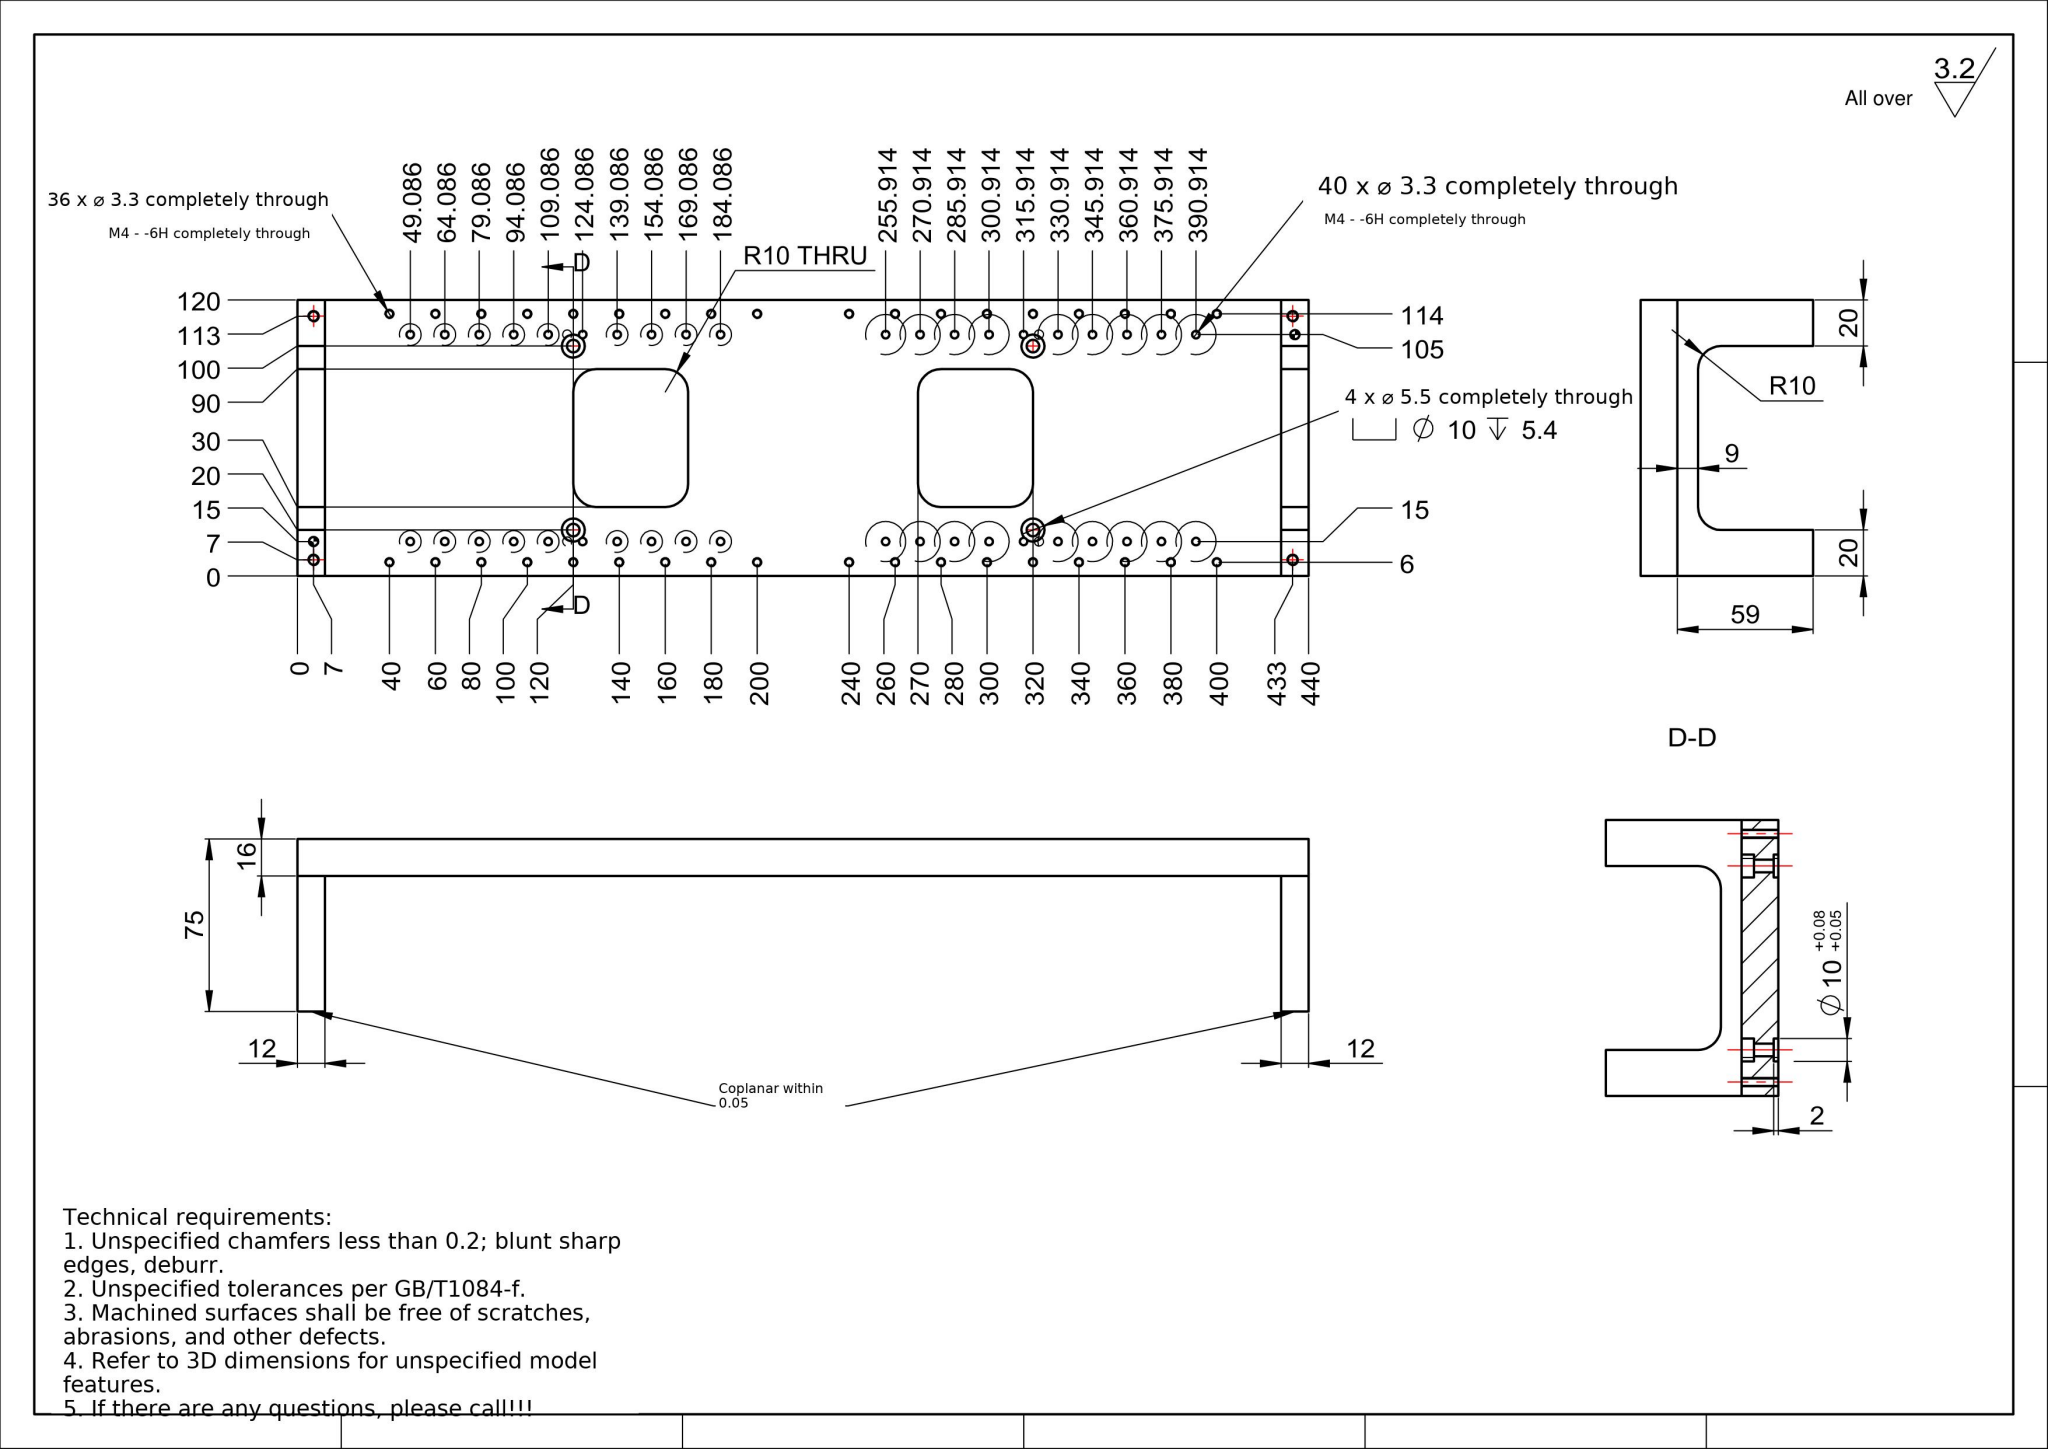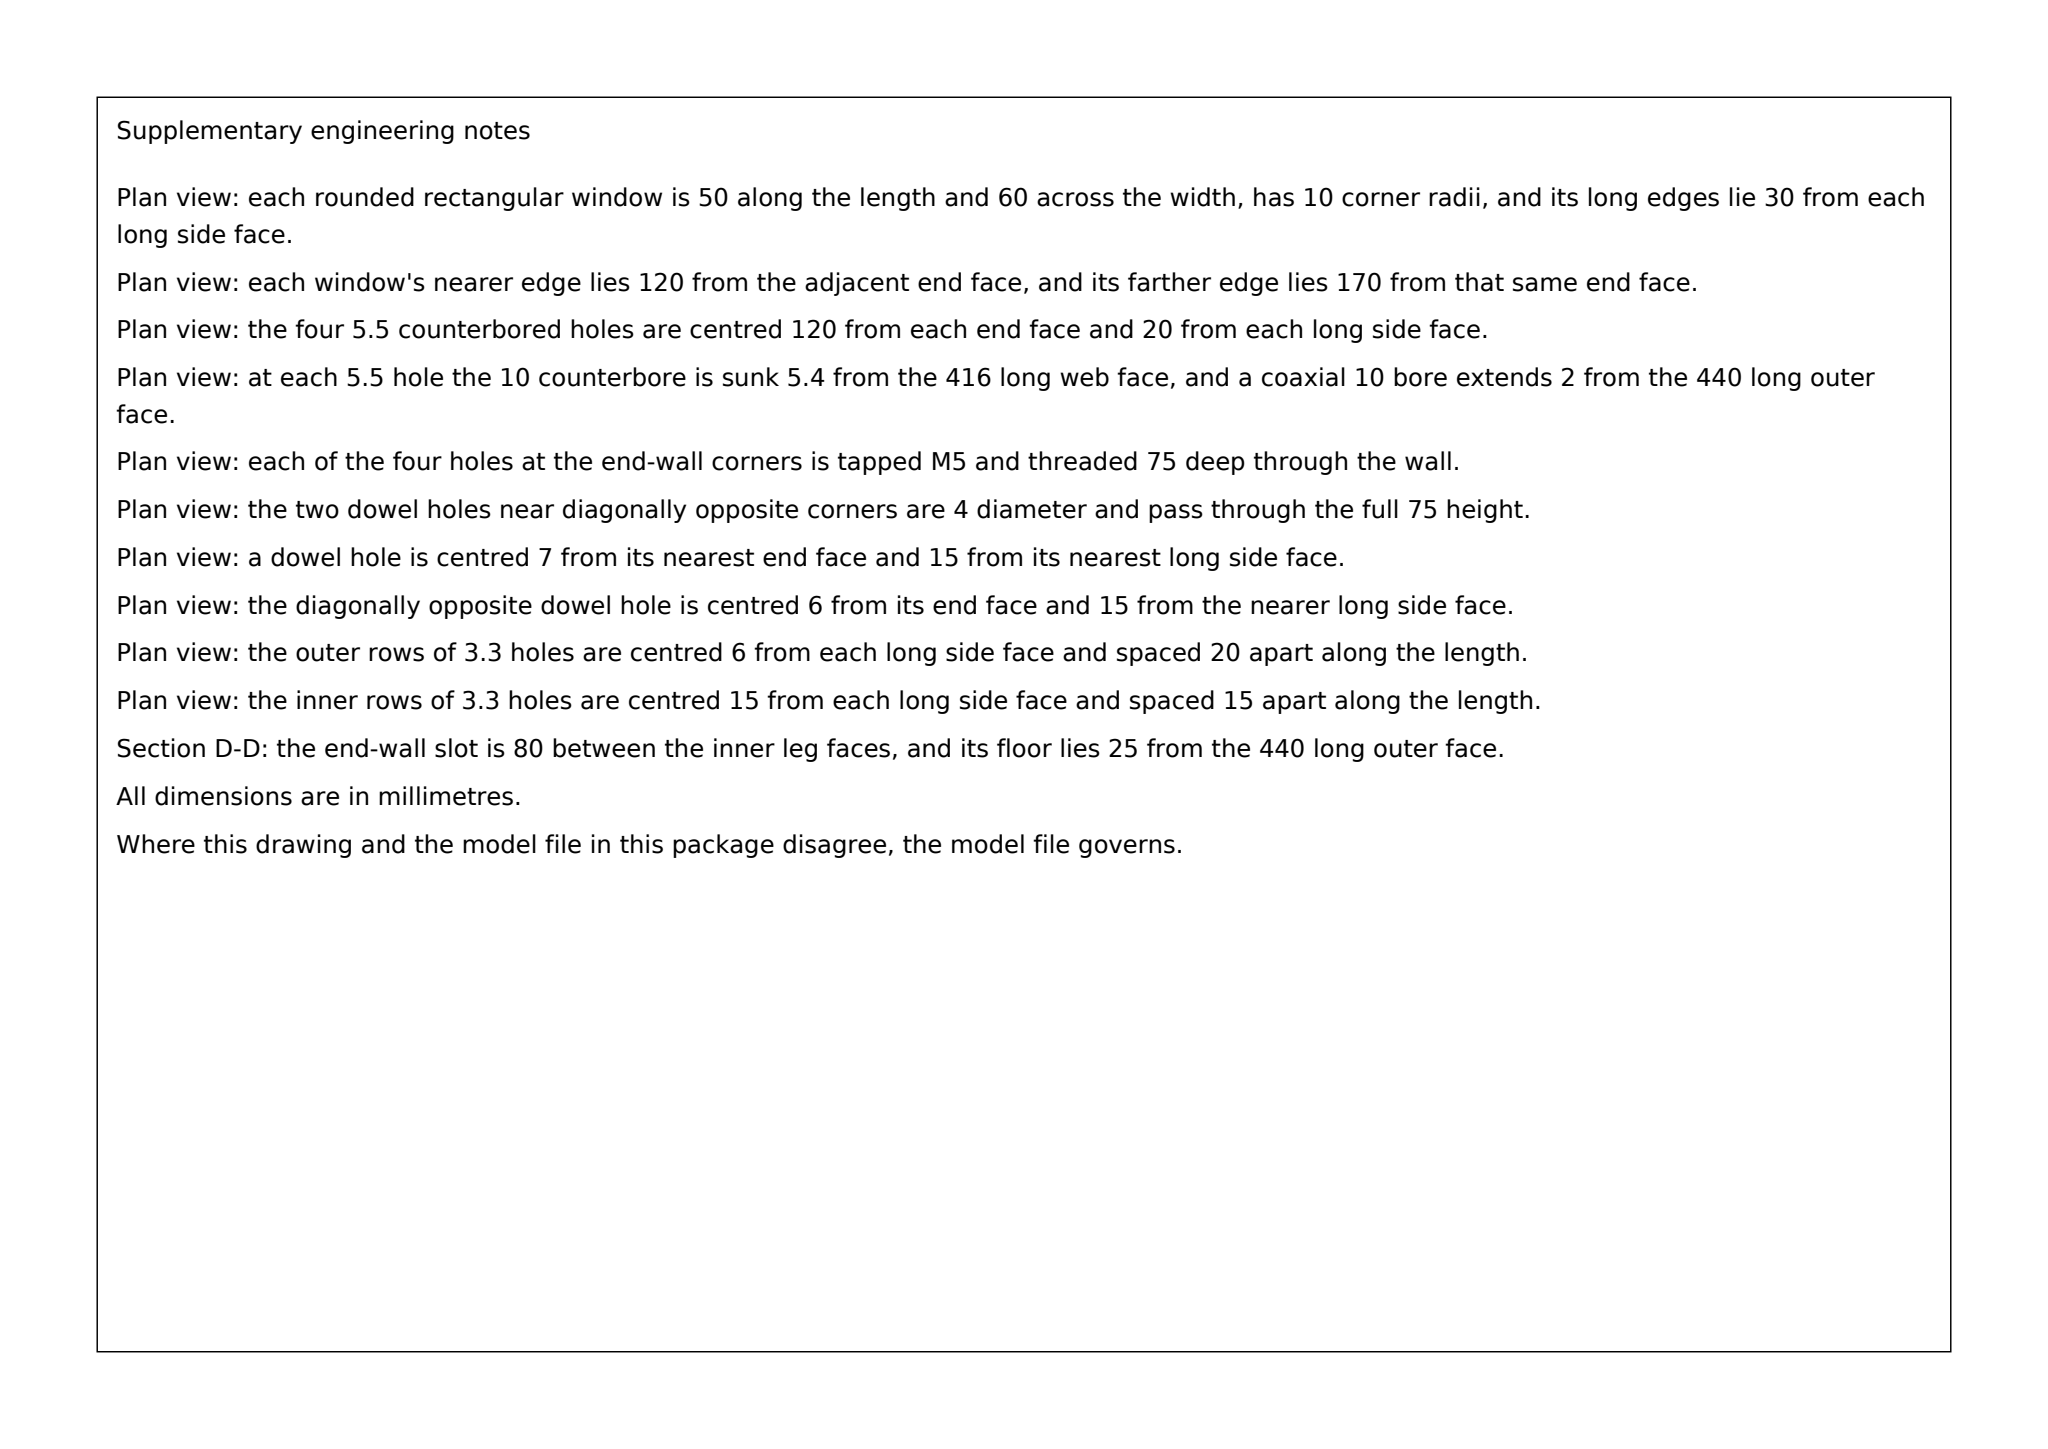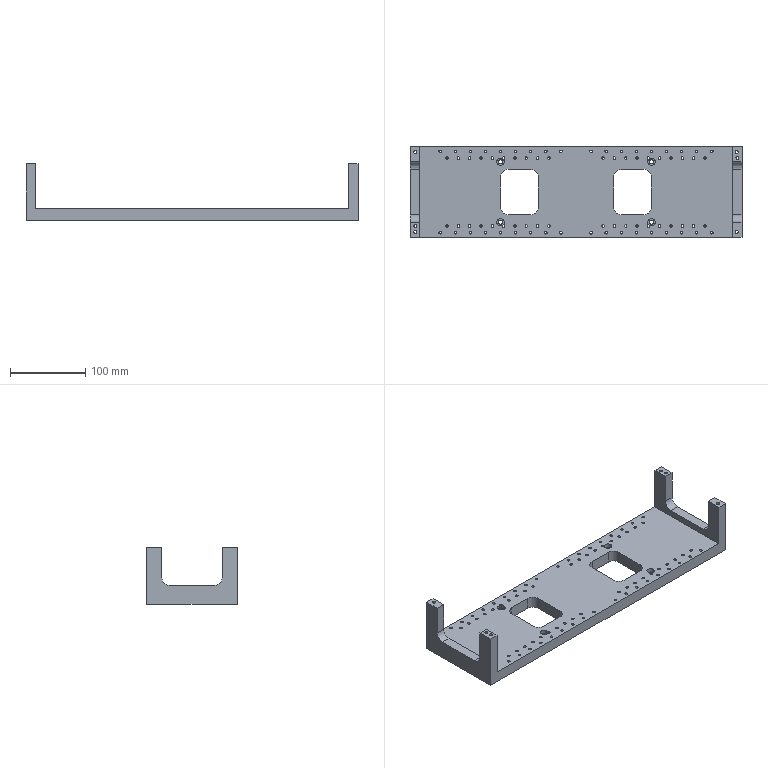Part | SolidWorks | mm | 1 solid | 242 faces | box 440 x 120 x 75 mm | volume 806918 mm3 | cylinder 208 | plane 34 | commonest cylinder face diameters 3.3 x152 10 x24 20 x12 5.5 x8 4.2 x8 4 x4
Drawing notes:
4X Ø4.2 THRU (full depth 75): two holes at x = 7, y = 7 and x = 7, y = 113, measured from the lower-left corner of the part (x0, y0). | from the solid: cylinders[4.2,z,[7.0,7.0],75.0] and cylinders[4.2,z,[7.0,113.0],75.0]
2X Ø4 THRU (full depth 75): one at x = 7, y = 15 and one at x = 434, y = 105 from the lower-left corner (x0, y0). | from the solid: cylinders[4.0,z,[7.0,15.0],75.0] and cylinders[4.0,z,[434.0,105.0],75.0]
R10 THRU pocket (left): pocket walls at x = 120 and x = 170 from the left end face (x = 0); right pocket walls at x = 270 and x = 320. | from the solid: axis_planes[x,120.0], [x,170.0], [x,270.0], [x,320.0]
4X Ø10 +0.08/+0.05 bore DP 2 deep, machined from the z = 0 face (opposite the Ø10 DP 5.4 counterbore face), coaxial with the 4X Ø5.5 THRU holes; counterbore floor at z = 10.6 from the z = 0 face. | from the solid: axis_planes[z,2.0]:count 4 and axis_planes[z,10.6]:count 4 (plate z = 0 to 16)
All dimensions are in millimetres; overall part envelope 440 x 120 x 75. | from the solid: bbox_xyz [440.0,120.0,75.0], STEP units mm
4X Ø4.2 THRU (full 75 height): 2 holes at X=7, Y=7 and 2 holes at X=7, Y=113, measured from the bbox min corner (X0/Y0/Z0 datum). | from the solid: cylinders [4.2,"z",[7.0,7.0],75.0,2] and [4.2,"z",[7.0,113.0],75.0,2]
2X Ø4 THRU (full 75 height): one at X=7, Y=15 and one at X=434, Y=105 from the X0/Y0 datum corner. | from the solid: cylinders [4.0,"z",[7.0,15.0],75.0,2] and [4.0,"z",[434.0,105.0],75.0,2]
Two R10-corner window cut-outs THRU: Y=30 to Y=90; first cut-out X=120 to X=170, second cut-out X=270 to X=320 from the X0/Y0 datum corner. | from the solid: axis_planes x 120.0/170.0/270.0/320.0 and y 30.0/90.0
Ø10 +0.08/+0.05 bore DP 2 in section D-D: 4 places, machined from the Z=0 face (bore floors at Z=2), i.e. opposite the Ø10 DP 5.4 counterbores which are machined from the Z=16 face (floors at Z=10.6). | from the solid: axis_planes ["z",2.0]:count 4 and ["z",10.6]:count 4 with ["z",0.0] and ["z",16.0] faces
All dimensions are in millimetres (mm). | from the solid: STEP model facts header: units mm